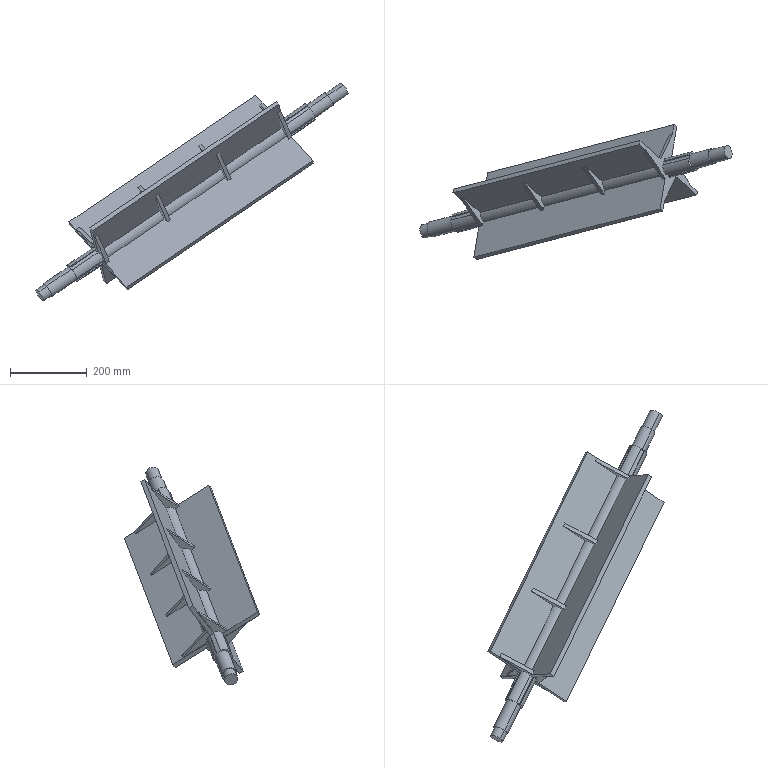Component | SolidWorks | CutterAxisI-1 | 1 solid | 119 faces | volume 4969008 mm3 | plane 91 | cylinder 28 | commonest cylinder face diameters 50 x20 35 x4 40 x4